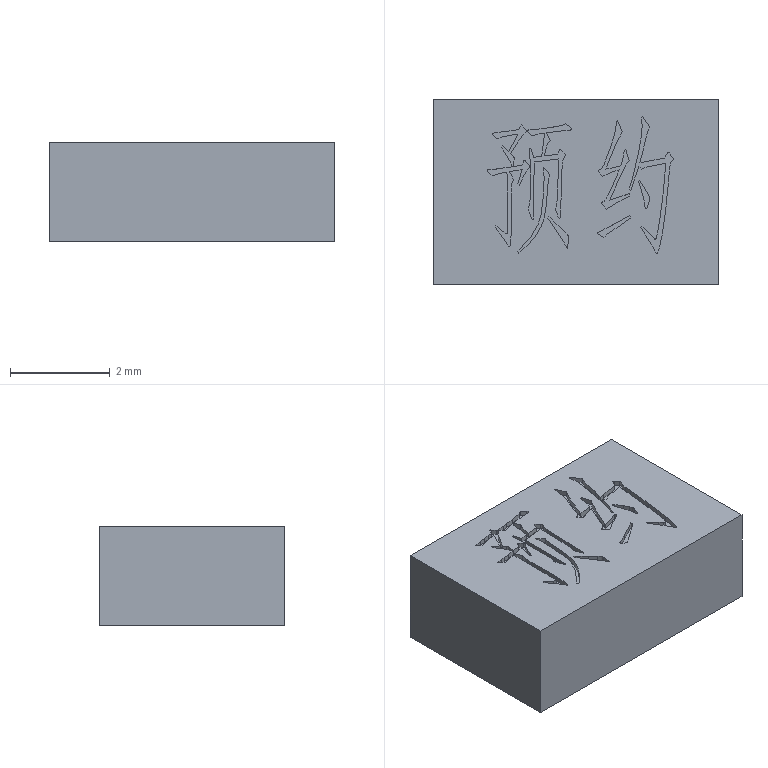Component | SolidWorks | Button4-1 | 1 solid | 206 faces | box 5.7 x 3.7 x 2 mm | volume 42 mm3 | plane 149 | spline 57
build123d program:
from build123d import *

# Parameters (mm, degrees)
SKETCH1_W           = 5.7
SKETCH1_H           = 3.7
BOSS_EXTRUDE1_DEPTH = 2
CUT_EXTRUDE1_DEPTH  = 0.1


with BuildPart() as part:
    # Sketch1 → Boss-Extrude1 (new body)
    with BuildSketch(Plane.XY):
        with Locations((2.85, 1.85)):
            Rectangle(SKETCH1_W, SKETCH1_H)
    extrude(amount=BOSS_EXTRUDE1_DEPTH)

    # Sketch2 → Cut-Extrude1 (cut)
    with BuildSketch(Plane.XY.offset(2)):
        with BuildLine():
            Line((1.574, 2.354), (1.551, 2.409))
            add(Edge.make_bspline(
                [(1.551, 2.409), (1.542, 2.43), (1.522, 2.474), (1.485, 2.54), (1.442, 2.612), (1.41, 2.66), (1.393, 2.685)],
                knots=[0, 0, 0, 0, 0.8687, 1.824, 2.865, 4, 4, 4, 4], degree=3))
            Line((1.393, 2.685), (1.359, 2.734))
            Line((1.359, 2.734), (1.373, 2.771))
            Line((1.373, 2.771), (1.396, 2.751))
            Line((1.396, 2.751), (1.505, 2.656))
            add(Edge.make_bspline(
                [(1.505, 2.656), (1.512, 2.667), (1.525, 2.69), (1.545, 2.727), (1.566, 2.766), (1.588, 2.808), (1.61, 2.854), (1.634, 2.902), (1.658, 2.953), (1.675, 2.989), (1.683, 3.007)],
                knots=[0, 0, 0, 0, 0.7801, 1.622, 2.525, 3.489, 4.524, 5.617, 6.775, 8, 8, 8, 8], degree=3))
            Line((1.683, 3.007), (1.577, 2.99))
            add(Edge.make_bspline(
                [(1.577, 2.99), (1.558, 2.987), (1.522, 2.98), (1.469, 2.97), (1.422, 2.961), (1.379, 2.952), (1.342, 2.942), (1.309, 2.933), (1.282, 2.924), (1.265, 2.918), (1.258, 2.915)],
                knots=[0, 0, 0, 0, 1.411, 2.709, 3.882, 4.944, 5.884, 6.704, 7.413, 8, 8, 8, 8], degree=3))
            Line((1.258, 2.915), (1.192, 2.987))
            add(Edge.make_bspline(
                [(1.192, 2.987), (1.186, 2.991), (1.178, 2.998), (1.172, 3.013), (1.179, 3.021), (1.189, 3.025), (1.204, 3.03), (1.216, 3.032), (1.223, 3.033)],
                knots=[0, 0, 0, 0, 1.454, 2.302, 2.76, 3.483, 4.56, 6, 6, 6, 6], degree=3))
            Line((1.223, 3.033), (1.353, 3.05))
            Line((1.353, 3.05), (1.485, 3.065))
            Line((1.485, 3.065), (1.591, 3.082))
            Line((1.591, 3.082), (1.701, 3.096))
            Line((1.701, 3.096), (1.741, 3.168))
            add(Edge.make_bspline(
                [(1.741, 3.168), (1.743, 3.172), (1.747, 3.179), (1.752, 3.187), (1.756, 3.192), (1.758, 3.196), (1.762, 3.194), (1.767, 3.19), (1.773, 3.183), (1.778, 3.177), (1.781, 3.174)],
                knots=[0, 0, 0, 0, 1.64, 2.878, 3.674, 4.05, 4.385, 5.107, 6.347, 8, 8, 8, 8], degree=3))
            Line((1.781, 3.174), (1.844, 3.099))
            add(Edge.make_bspline(
                [(1.844, 3.099), (1.849, 3.093), (1.855, 3.083), (1.859, 3.068), (1.855, 3.058), (1.849, 3.05), (1.839, 3.041), (1.821, 3.027), (1.795, 3.003), (1.773, 2.975), (1.754, 2.949), (1.739, 2.926), (1.718, 2.895), (1.693, 2.855), (1.662, 2.808), (1.625, 2.752), (1.585, 2.688), (1.555, 2.643), (1.54, 2.619)],
                knots=[0, 0, 0, 0, 0.5778, 0.9885, 1.187, 1.454, 1.816, 2.262, 3.348, 4.677, 5.177, 5.931, 6.952, 8.228, 9.781, 11.595, 13.664, 16, 16, 16, 16], degree=3))
            Line((1.54, 2.619), (1.597, 2.558))
            add(Edge.make_bspline(
                [(1.597, 2.558), (1.6, 2.554), (1.605, 2.546), (1.611, 2.537), (1.613, 2.529), (1.612, 2.519), (1.611, 2.506), (1.61, 2.495), (1.609, 2.489)],
                knots=[0, 0, 0, 0, 1.384, 2.211, 2.635, 3.368, 4.524, 6, 6, 6, 6], degree=3))
            Line((1.609, 2.489), (1.586, 2.357))
            Line((1.586, 2.357), (1.767, 2.383))
            Line((1.767, 2.383), (1.801, 2.461))
            add(Edge.make_bspline(
                [(1.801, 2.461), (1.804, 2.465), (1.807, 2.473), (1.82, 2.48), (1.834, 2.473), (1.84, 2.465), (1.844, 2.461)],
                knots=[0, 0, 0, 0, 1.058, 1.818, 2.714, 4, 4, 4, 4], degree=3))
            Line((1.844, 2.461), (1.896, 2.394))
            add(Edge.make_bspline(
                [(1.896, 2.394), (1.9, 2.389), (1.906, 2.379), (1.913, 2.367), (1.917, 2.357), (1.919, 2.349), (1.915, 2.342), (1.908, 2.332), (1.898, 2.32), (1.883, 2.305), (1.866, 2.284), (1.847, 2.256), (1.826, 2.22), (1.812, 2.193), (1.804, 2.179)],
                knots=[0, 0, 0, 0, 0.87, 1.559, 2.026, 2.348, 2.671, 3.202, 3.926, 4.901, 6.149, 7.717, 9.686, 12, 12, 12, 12], degree=3))
            Line((1.804, 2.179), (1.761, 2.081))
            Line((1.761, 2.081), (1.712, 1.977))
            Line((1.712, 1.977), (1.686, 2.009))
            Line((1.686, 2.009), (1.773, 2.297))
            Line((1.773, 2.297), (1.514, 2.256))
            Line((1.514, 2.256), (1.6, 2.106))
            add(Edge.make_bspline(
                [(1.6, 2.106), (1.596, 2.095), (1.587, 2.075), (1.576, 2.049), (1.57, 2.029), (1.565, 2.015), (1.564, 2), (1.563, 1.981), (1.561, 1.956), (1.56, 1.936), (1.56, 1.925)],
                knots=[0, 0, 0, 0, 1.554, 2.768, 3.652, 4.198, 4.709, 5.51, 6.619, 8, 8, 8, 8], degree=3))
            Line((1.56, 1.925), (1.554, 1.828))
            Line((1.554, 1.828), (1.551, 1.117))
            Line((1.551, 1.117), (1.551, 1.013))
            add(Edge.make_bspline(
                [(1.551, 1.013), (1.55, 0.9875), (1.548, 0.9319), (1.543, 0.8624), (1.538, 0.8088), (1.533, 0.778), (1.528, 0.7589), (1.519, 0.747), (1.509, 0.7499), (1.5, 0.7564), (1.49, 0.7675), (1.477, 0.7866), (1.464, 0.8099), (1.455, 0.8278), (1.451, 0.8352)],
                knots=[0, 0, 0, 0, 2.434, 5.233, 6.549, 7.511, 8.132, 8.453, 8.71, 9.047, 9.501, 10.086, 11.211, 12, 12, 12, 12], degree=3))
            Line((1.451, 0.8352), (1.353, 0.9818))
            Line((1.353, 0.9818), (1.232, 1.14))
            Line((1.232, 1.14), (1.246, 1.177))
            Line((1.246, 1.177), (1.405, 1.048))
            add(Edge.make_bspline(
                [(1.405, 1.048), (1.412, 1.042), (1.423, 1.032), (1.44, 1.021), (1.452, 1.014), (1.463, 1.014), (1.469, 1.023), (1.471, 1.036), (1.473, 1.055), (1.472, 1.089), (1.471, 1.139), (1.473, 1.207), (1.476, 1.281), (1.478, 1.332), (1.479, 1.359)],
                knots=[0, 0, 0, 0, 0.7812, 1.36, 1.741, 1.977, 2.215, 2.595, 3.128, 3.832, 5.549, 7.538, 9.714, 12, 12, 12, 12], degree=3))
            Line((1.479, 1.359), (1.482, 1.848))
            add(Edge.make_bspline(
                [(1.482, 1.848), (1.482, 1.869), (1.482, 1.907), (1.482, 1.962), (1.482, 2.008), (1.481, 2.047), (1.48, 2.079), (1.479, 2.105), (1.479, 2.126), (1.478, 2.143), (1.476, 2.16), (1.473, 2.183), (1.47, 2.211), (1.467, 2.233), (1.465, 2.245)],
                knots=[0, 0, 0, 0, 1.878, 3.511, 4.913, 6.071, 7.023, 7.82, 8.438, 8.889, 9.366, 10.039, 10.921, 12, 12, 12, 12], degree=3))
            Line((1.465, 2.245), (1.353, 2.228))
            add(Edge.make_bspline(
                [(1.353, 2.228), (1.321, 2.221), (1.258, 2.208), (1.199, 2.185), (1.169, 2.173)],
                knots=[0, 0, 0, 0, 0.9976, 2, 2, 2, 2], degree=3))
            Line((1.169, 2.173), (1.083, 2.256))
            add(Edge.make_bspline(
                [(1.083, 2.256), (1.078, 2.26), (1.071, 2.267), (1.069, 2.283), (1.085, 2.292), (1.096, 2.293), (1.103, 2.294)],
                knots=[0, 0, 0, 0, 1.139, 1.841, 2.65, 4, 4, 4, 4], degree=3))
            Line((1.103, 2.294), (1.192, 2.302))
            Line((1.192, 2.302), (1.284, 2.311))
            Line((1.284, 2.311), (1.428, 2.334))
            Line((1.428, 2.334), (1.574, 2.354))
        make_face()
        with BuildLine():
            Line((1.681, 0.6656), (1.715, 0.7001))
            add(Edge.make_bspline(
                [(1.715, 0.7001), (1.734, 0.7193), (1.769, 0.7556), (1.819, 0.8079), (1.862, 0.855), (1.901, 0.898), (1.938, 0.9442), (1.975, 0.9977), (2.014, 1.061), (2.054, 1.131), (2.092, 1.205), (2.123, 1.282), (2.145, 1.357), (2.159, 1.434), (2.168, 1.514), (2.178, 1.598), (2.188, 1.689), (2.197, 1.784), (2.205, 1.88), (2.21, 1.971), (2.213, 2.055), (2.213, 2.109), (2.213, 2.135)],
                knots=[0, 0, 0, 0, 1.017, 1.931, 2.738, 3.443, 4.154, 4.978, 5.915, 6.968, 8.056, 9.097, 10.095, 11.063, 12.06, 13.137, 14.301, 15.539, 16.781, 17.94, 19.011, 20, 20, 20, 20], degree=3))
            add(Edge.make_bspline(
                [(2.213, 2.135), (2.212, 2.147), (2.212, 2.169), (2.209, 2.199), (2.208, 2.225), (2.205, 2.241), (2.204, 2.248)],
                knots=[0, 0, 0, 0, 1.244, 2.322, 3.25, 4, 4, 4, 4], degree=3))
            Line((2.204, 2.248), (2.196, 2.311))
            Line((2.196, 2.311), (2.204, 2.343))
            Line((2.204, 2.343), (2.325, 2.196))
            add(Edge.make_bspline(
                [(2.325, 2.196), (2.322, 2.187), (2.315, 2.17), (2.306, 2.143), (2.299, 2.111), (2.294, 2.083), (2.292, 2.058), (2.29, 2.04), (2.288, 2.018), (2.287, 1.992), (2.285, 1.962), (2.283, 1.928), (2.281, 1.89), (2.278, 1.833), (2.274, 1.757), (2.265, 1.663), (2.254, 1.564), (2.241, 1.463), (2.223, 1.362), (2.195, 1.264), (2.16, 1.171), (2.115, 1.084), (2.066, 1.003), (2.014, 0.9282), (1.96, 0.8607), (1.904, 0.802), (1.851, 0.7519), (1.806, 0.7092), (1.768, 0.6751), (1.745, 0.6563), (1.735, 0.6481)],
                knots=[0, 0, 0, 0, 0.4735, 0.8985, 1.382, 2.069, 2.292, 2.584, 2.945, 3.369, 3.855, 4.41, 5.034, 5.721, 7.193, 8.737, 10.347, 12.024, 13.709, 15.35, 16.968, 18.567, 20.121, 21.589, 22.993, 24.326, 25.536, 26.551, 27.37, 28, 28, 28, 28], degree=3))
            Line((1.735, 0.6481), (1.701, 0.6221))
            Line((1.701, 0.6221), (1.681, 0.6656))
        make_face()
        with BuildLine():
            Line((2.15, 3.114), (2.334, 3.14))
            add(Edge.make_bspline(
                [(2.334, 3.14), (2.353, 3.142), (2.388, 3.148), (2.438, 3.156), (2.482, 3.163), (2.519, 3.17), (2.55, 3.178), (2.575, 3.184), (2.593, 3.19), (2.603, 3.195), (2.607, 3.197)],
                knots=[0, 0, 0, 0, 1.638, 3.081, 4.354, 5.434, 6.346, 7.076, 7.619, 8, 8, 8, 8], degree=3))
            Line((2.607, 3.197), (2.647, 3.22))
            Line((2.647, 3.22), (2.748, 3.137))
            add(Edge.make_bspline(
                [(2.748, 3.137), (2.753, 3.131), (2.763, 3.123), (2.769, 3.108), (2.766, 3.097), (2.758, 3.093), (2.747, 3.089), (2.739, 3.088), (2.733, 3.088)],
                knots=[0, 0, 0, 0, 1.676, 2.889, 3.395, 3.99, 4.869, 6, 6, 6, 6], degree=3))
            Line((2.733, 3.088), (2.48, 3.062))
            Line((2.48, 3.062), (2.256, 3.033))
            Line((2.256, 3.033), (2.331, 2.889))
            add(Edge.make_bspline(
                [(2.331, 2.889), (2.323, 2.879), (2.306, 2.856), (2.287, 2.828), (2.273, 2.804), (2.267, 2.785), (2.259, 2.761), (2.251, 2.733), (2.243, 2.699), (2.235, 2.66), (2.227, 2.617), (2.221, 2.586), (2.219, 2.57)],
                knots=[0, 0, 0, 0, 1.092, 2.497, 2.946, 3.532, 4.25, 5.111, 6.12, 7.273, 8.563, 10, 10, 10, 10], degree=3))
            Line((2.219, 2.57), (2.486, 2.604))
            Line((2.486, 2.604), (2.512, 2.679))
            add(Edge.make_bspline(
                [(2.512, 2.679), (2.514, 2.684), (2.518, 2.693), (2.525, 2.703), (2.534, 2.708), (2.539, 2.704), (2.541, 2.702)],
                knots=[0, 0, 0, 0, 1.53, 2.568, 3.261, 4, 4, 4, 4], degree=3))
            Line((2.541, 2.702), (2.613, 2.624))
            add(Edge.make_bspline(
                [(2.613, 2.624), (2.619, 2.617), (2.629, 2.605), (2.639, 2.585), (2.634, 2.565), (2.626, 2.553), (2.621, 2.547)],
                knots=[0, 0, 0, 0, 1.29, 2.137, 2.904, 4, 4, 4, 4], degree=3))
            add(Edge.make_bspline(
                [(2.621, 2.547), (2.614, 2.536), (2.601, 2.516), (2.588, 2.489), (2.581, 2.464), (2.577, 2.442), (2.574, 2.415), (2.573, 2.396), (2.572, 2.386)],
                knots=[0, 0, 0, 0, 1.308, 2.536, 3.188, 3.978, 4.923, 6, 6, 6, 6], degree=3))
            Line((2.572, 2.386), (2.549, 1.687))
            add(Edge.make_bspline(
                [(2.549, 1.687), (2.549, 1.663), (2.547, 1.62), (2.545, 1.561), (2.544, 1.515), (2.542, 1.48), (2.541, 1.449), (2.539, 1.417), (2.535, 1.382), (2.533, 1.352), (2.53, 1.329), (2.527, 1.318), (2.523, 1.309), (2.515, 1.31), (2.51, 1.317), (2.504, 1.329), (2.496, 1.346), (2.491, 1.36), (2.489, 1.368)],
                knots=[0, 0, 0, 0, 2.539, 4.638, 6.264, 7.451, 8.454, 9.581, 10.848, 12.222, 12.837, 13.265, 13.526, 13.693, 13.994, 14.464, 15.13, 16, 16, 16, 16], degree=3))
            Line((2.489, 1.368), (2.454, 1.465))
            add(Edge.make_bspline(
                [(2.454, 1.465), (2.452, 1.472), (2.448, 1.484), (2.443, 1.499), (2.439, 1.51), (2.438, 1.519), (2.445, 1.532), (2.451, 1.554), (2.46, 1.586), (2.466, 1.623), (2.471, 1.659), (2.476, 1.687), (2.478, 1.71), (2.48, 1.731), (2.48, 1.757), (2.48, 1.777), (2.48, 1.787)],
                knots=[0, 0, 0, 0, 0.9227, 1.61, 2.081, 2.299, 2.815, 3.846, 5.275, 6.985, 8.668, 9.952, 10.626, 11.517, 12.641, 14, 14, 14, 14], degree=3))
            Line((2.48, 1.787), (2.489, 2.069))
            Line((2.489, 2.069), (2.5, 2.509))
            Line((2.5, 2.509), (2.012, 2.449))
            Line((2.012, 2.449), (2.003, 1.557))
            Line((2.003, 1.557), (2, 1.353))
            add(Edge.make_bspline(
                [(2, 1.353), (2, 1.346), (2, 1.335), (1.998, 1.319), (1.996, 1.308), (1.991, 1.299), (1.984, 1.293), (1.975, 1.293), (1.971, 1.299), (1.967, 1.307), (1.962, 1.319), (1.959, 1.328), (1.957, 1.333)],
                knots=[0, 0, 0, 0, 1.685, 3.012, 3.999, 4.703, 5.59, 6.251, 6.743, 7.53, 8.598, 10, 10, 10, 10], degree=3))
            Line((1.957, 1.333), (1.914, 1.442))
            add(Edge.make_bspline(
                [(1.914, 1.442), (1.91, 1.45), (1.903, 1.464), (1.896, 1.482), (1.891, 1.494), (1.889, 1.502), (1.891, 1.507), (1.893, 1.515), (1.897, 1.525), (1.905, 1.543), (1.914, 1.573), (1.921, 1.616), (1.928, 1.661), (1.931, 1.708), (1.934, 1.76), (1.936, 1.796), (1.937, 1.816)],
                knots=[0, 0, 0, 0, 0.9721, 1.681, 2.148, 2.367, 2.529, 2.809, 3.207, 3.708, 5.009, 6.634, 8.387, 10.007, 11.795, 14, 14, 14, 14], degree=3))
            Line((1.937, 1.816), (1.937, 2.394))
            add(Edge.make_bspline(
                [(1.937, 2.394), (1.937, 2.395), (1.937, 2.398), (1.937, 2.405), (1.937, 2.416), (1.937, 2.432), (1.936, 2.452), (1.936, 2.478), (1.934, 2.508), (1.932, 2.558), (1.927, 2.628), (1.92, 2.686), (1.917, 2.716)],
                knots=[0, 0, 0, 0, 0.06597, 0.2771, 0.6201, 1.108, 1.742, 2.547, 3.485, 4.594, 7.134, 10, 10, 10, 10], degree=3))
            Line((1.917, 2.716), (1.945, 2.728))
            Line((1.945, 2.728), (2.003, 2.541))
            Line((2.003, 2.541), (2.164, 2.564))
            add(Edge.make_bspline(
                [(2.164, 2.564), (2.167, 2.581), (2.172, 2.612), (2.179, 2.651), (2.184, 2.686), (2.189, 2.719), (2.193, 2.762), (2.199, 2.81), (2.204, 2.856), (2.207, 2.895), (2.209, 2.923), (2.21, 2.938), (2.21, 2.944)],
                knots=[0, 0, 0, 0, 1.298, 2.473, 3.138, 4.037, 5.146, 6.49, 7.8, 8.828, 9.554, 10, 10, 10, 10], degree=3))
            Line((2.21, 2.944), (2.213, 3.027))
            add(Edge.make_bspline(
                [(2.213, 3.027), (2.189, 3.024), (2.144, 3.018), (2.08, 3.005), (2.022, 2.99), (1.986, 2.976), (1.969, 2.969)],
                knots=[0, 0, 0, 0, 1.129, 2.166, 3.121, 4, 4, 4, 4], degree=3))
            Line((1.969, 2.969), (1.891, 3.047))
            add(Edge.make_bspline(
                [(1.891, 3.047), (1.887, 3.052), (1.88, 3.059), (1.874, 3.071), (1.876, 3.08), (1.883, 3.084), (1.894, 3.088), (1.903, 3.089), (1.908, 3.091)],
                knots=[0, 0, 0, 0, 1.498, 2.59, 3.084, 3.731, 4.696, 6, 6, 6, 6], degree=3))
            Line((1.908, 3.091), (2.038, 3.102))
            Line((2.038, 3.102), (2.15, 3.114))
        make_face()
        with BuildLine():
            Line((2.285, 1.327), (2.305, 1.365))
            Line((2.305, 1.365), (2.36, 1.31))
            Line((2.36, 1.31), (2.512, 1.16))
            Line((2.512, 1.16), (2.647, 1.028))
            add(Edge.make_bspline(
                [(2.647, 1.028), (2.653, 1.022), (2.663, 1.011), (2.676, 0.9954), (2.686, 0.9836), (2.695, 0.9711), (2.701, 0.9521), (2.7, 0.9364), (2.699, 0.9273)],
                knots=[0, 0, 0, 0, 1.256, 2.285, 3.069, 3.615, 4.615, 6, 6, 6, 6], degree=3))
            Line((2.699, 0.9273), (2.687, 0.7777))
            add(Edge.make_bspline(
                [(2.687, 0.7777), (2.687, 0.7717), (2.686, 0.7612), (2.685, 0.7477), (2.684, 0.7388), (2.684, 0.7328), (2.68, 0.7288), (2.675, 0.7256), (2.668, 0.7315), (2.661, 0.7416), (2.652, 0.759), (2.645, 0.7727), (2.641, 0.7807)],
                knots=[0, 0, 0, 0, 1.5, 2.645, 3.397, 3.76, 4.117, 4.659, 5.124, 6.143, 7.769, 10, 10, 10, 10], degree=3))
            Line((2.641, 0.7807), (2.601, 0.8523))
            add(Edge.make_bspline(
                [(2.601, 0.8523), (2.594, 0.8651), (2.579, 0.8922), (2.553, 0.9347), (2.523, 0.9812), (2.49, 1.033), (2.453, 1.088), (2.412, 1.148), (2.367, 1.211), (2.335, 1.255), (2.319, 1.278)],
                knots=[0, 0, 0, 0, 0.6936, 1.466, 2.336, 3.291, 4.335, 5.467, 6.689, 8, 8, 8, 8], degree=3))
            Line((2.319, 1.278), (2.285, 1.327))
        make_face()
        with BuildLine():
            Line((3.915, 1.905), (3.929, 1.954))
            Line((3.929, 1.954), (3.969, 2.083))
            add(Edge.make_bspline(
                [(3.969, 2.083), (3.972, 2.092), (3.977, 2.11), (3.985, 2.14), (3.993, 2.174), (4.003, 2.212), (4.013, 2.255), (4.025, 2.302), (4.037, 2.354), (4.05, 2.409), (4.063, 2.463), (4.075, 2.515), (4.085, 2.563), (4.095, 2.606), (4.103, 2.645), (4.111, 2.68), (4.117, 2.71), (4.126, 2.761), (4.138, 2.835), (4.151, 2.915), (4.16, 2.976), (4.165, 3.016), (4.17, 3.049), (4.173, 3.086), (4.176, 3.127), (4.176, 3.158), (4.176, 3.174)],
                knots=[0, 0, 0, 0, 0.5622, 1.229, 1.988, 2.842, 3.788, 4.838, 5.983, 7.23, 8.477, 9.619, 10.675, 11.634, 12.491, 13.261, 13.927, 14.506, 16.624, 18.747, 19.751, 20.614, 21.346, 21.946, 22.988, 24, 24, 24, 24], degree=3))
            add(Edge.make_bspline(
                [(4.176, 3.174), (4.176, 3.186), (4.174, 3.21), (4.17, 3.248), (4.164, 3.289), (4.159, 3.317), (4.156, 3.332)],
                knots=[0, 0, 0, 0, 0.8682, 1.824, 2.872, 4, 4, 4, 4], degree=3))
            Line((4.156, 3.332), (4.176, 3.361))
            Line((4.176, 3.361), (4.326, 3.154))
            add(Edge.make_bspline(
                [(4.326, 3.154), (4.319, 3.139), (4.306, 3.112), (4.29, 3.071), (4.276, 3.033), (4.265, 2.995), (4.256, 2.957), (4.246, 2.914), (4.234, 2.867), (4.223, 2.816), (4.211, 2.765), (4.2, 2.719), (4.191, 2.678), (4.185, 2.653), (4.182, 2.642)],
                knots=[0, 0, 0, 0, 1.078, 2.063, 2.979, 3.817, 4.676, 5.654, 6.759, 7.981, 9.193, 10.266, 11.202, 12, 12, 12, 12], degree=3))
            Line((4.182, 2.642), (4.145, 2.498))
            Line((4.145, 2.498), (4.13, 2.438))
            Line((4.13, 2.438), (4.243, 2.455))
            Line((4.243, 2.455), (4.619, 2.527))
            Line((4.619, 2.527), (4.674, 2.624))
            add(Edge.make_bspline(
                [(4.674, 2.624), (4.678, 2.63), (4.683, 2.64), (4.697, 2.648), (4.713, 2.643), (4.719, 2.635), (4.723, 2.63)],
                knots=[0, 0, 0, 0, 1.227, 2.09, 2.863, 4, 4, 4, 4], degree=3))
            Line((4.723, 2.63), (4.78, 2.544))
            add(Edge.make_bspline(
                [(4.78, 2.544), (4.783, 2.54), (4.788, 2.532), (4.793, 2.522), (4.796, 2.514), (4.797, 2.508), (4.793, 2.502), (4.789, 2.495), (4.781, 2.485), (4.768, 2.469), (4.753, 2.45), (4.742, 2.429), (4.737, 2.41), (4.733, 2.391), (4.73, 2.364), (4.727, 2.345), (4.726, 2.334)],
                knots=[0, 0, 0, 0, 0.9006, 1.591, 2.08, 2.39, 2.701, 3.244, 3.98, 4.949, 6.88, 8.376, 9.207, 10.414, 12.027, 14, 14, 14, 14], degree=3))
            Line((4.726, 2.334), (4.711, 2.176))
            Line((4.711, 2.176), (4.688, 1.922))
            Line((4.688, 1.922), (4.657, 1.609))
            Line((4.657, 1.609), (4.625, 1.336))
            Line((4.625, 1.336), (4.608, 1.215))
            Line((4.608, 1.215), (4.585, 1.051))
            add(Edge.make_bspline(
                [(4.585, 1.051), (4.583, 1.038), (4.577, 1.009), (4.568, 0.9614), (4.557, 0.9029), (4.545, 0.849), (4.536, 0.8039), (4.529, 0.7724), (4.523, 0.7441), (4.516, 0.7193), (4.511, 0.6976), (4.505, 0.6797), (4.501, 0.6647), (4.495, 0.6504), (4.489, 0.6366), (4.481, 0.624), (4.475, 0.6156), (4.469, 0.6109), (4.462, 0.6136), (4.456, 0.6207), (4.45, 0.6313), (4.446, 0.6401), (4.444, 0.6452)],
                knots=[0, 0, 0, 0, 1.538, 3.495, 5.869, 8.664, 10.088, 11.375, 12.526, 13.561, 14.439, 15.203, 15.811, 16.307, 17.06, 17.631, 18.043, 18.294, 18.525, 18.85, 19.346, 20, 20, 20, 20], degree=3))
            Line((4.444, 0.6452), (4.392, 0.7432))
            Line((4.392, 0.7432), (4.323, 0.8612))
            Line((4.323, 0.8612), (4.15, 1.134))
            Line((4.15, 1.134), (4.171, 1.166))
            Line((4.171, 1.166), (4.263, 1.074))
            Line((4.263, 1.074), (4.343, 0.9933))
            Line((4.343, 0.9933), (4.401, 0.9328))
            add(Edge.make_bspline(
                [(4.401, 0.9328), (4.405, 0.9286), (4.411, 0.921), (4.422, 0.9128), (4.429, 0.9068), (4.438, 0.9046), (4.446, 0.9096), (4.454, 0.9203), (4.459, 0.9384), (4.462, 0.953), (4.464, 0.9618)],
                knots=[0, 0, 0, 0, 1.23, 2.183, 2.844, 3.281, 3.99, 4.796, 6.06, 8, 8, 8, 8], degree=3))
            Line((4.464, 0.9618), (4.481, 1.028))
            Line((4.481, 1.028), (4.504, 1.149))
            Line((4.504, 1.149), (4.53, 1.31))
            Line((4.53, 1.31), (4.562, 1.557))
            Line((4.562, 1.557), (4.591, 1.787))
            Line((4.591, 1.787), (4.614, 2.043))
            Line((4.614, 2.043), (4.637, 2.291))
            Line((4.637, 2.291), (4.645, 2.423))
            add(Edge.make_bspline(
                [(4.645, 2.423), (4.622, 2.418), (4.575, 2.408), (4.508, 2.395), (4.445, 2.384), (4.384, 2.374), (4.326, 2.364), (4.27, 2.349), (4.215, 2.332), (4.18, 2.316), (4.162, 2.308)],
                knots=[0, 0, 0, 0, 1.168, 2.269, 3.304, 4.275, 5.208, 6.134, 7.065, 8, 8, 8, 8], degree=3))
            Line((4.162, 2.308), (4.107, 2.36))
            add(Edge.make_bspline(
                [(4.107, 2.36), (4.101, 2.339), (4.088, 2.299), (4.07, 2.242), (4.053, 2.19), (4.038, 2.145), (4.025, 2.104), (4.013, 2.07), (4.004, 2.041), (3.993, 2.011), (3.983, 1.982), (3.973, 1.954), (3.966, 1.934), (3.962, 1.924), (3.961, 1.92)],
                knots=[0, 0, 0, 0, 1.702, 3.255, 4.646, 5.899, 6.99, 7.932, 8.724, 9.366, 10.371, 11.141, 11.693, 12, 12, 12, 12], degree=3))
            Line((3.961, 1.92), (3.949, 1.879))
            Line((3.949, 1.879), (3.915, 1.905))
        make_face()
        with BuildLine():
            Line((4.101, 2.055), (4.122, 2.086))
            Line((4.122, 2.086), (4.15, 2.046))
            Line((4.15, 2.046), (4.24, 1.905))
            Line((4.24, 1.905), (4.309, 1.782))
            add(Edge.make_bspline(
                [(4.309, 1.782), (4.313, 1.771), (4.32, 1.753), (4.328, 1.727), (4.329, 1.7), (4.323, 1.684), (4.32, 1.675)],
                knots=[0, 0, 0, 0, 1.204, 2.145, 2.991, 4, 4, 4, 4], degree=3))
            Line((4.32, 1.675), (4.272, 1.534))
            add(Edge.make_bspline(
                [(4.272, 1.534), (4.269, 1.528), (4.266, 1.519), (4.257, 1.507), (4.244, 1.509), (4.24, 1.516), (4.237, 1.52)],
                knots=[0, 0, 0, 0, 1.411, 2.275, 2.954, 4, 4, 4, 4], degree=3))
            Line((4.237, 1.52), (4.225, 1.606))
            Line((4.225, 1.606), (4.197, 1.753))
            add(Edge.make_bspline(
                [(4.197, 1.753), (4.195, 1.761), (4.19, 1.78), (4.183, 1.808), (4.174, 1.841), (4.163, 1.877), (4.15, 1.916), (4.135, 1.96), (4.119, 2.006), (4.107, 2.038), (4.101, 2.055)],
                knots=[0, 0, 0, 0, 0.6627, 1.419, 2.268, 3.224, 4.265, 5.411, 6.663, 8, 8, 8, 8], degree=3))
        make_face()
        with BuildLine():
            add(Edge.make_bspline(
                [(3.446, 2.305), (3.469, 2.31), (3.516, 2.319), (3.59, 2.334), (3.666, 2.352), (3.718, 2.365), (3.745, 2.371)],
                knots=[0, 0, 0, 0, 0.9252, 1.903, 2.925, 4, 4, 4, 4], degree=3))
            Line((3.745, 2.371), (3.774, 2.458))
            add(Edge.make_bspline(
                [(3.774, 2.458), (3.775, 2.462), (3.778, 2.472), (3.781, 2.49), (3.787, 2.512), (3.792, 2.538), (3.798, 2.563), (3.802, 2.584), (3.806, 2.599), (3.808, 2.607), (3.808, 2.61)],
                knots=[0, 0, 0, 0, 0.6556, 1.592, 2.776, 4.225, 5.653, 6.747, 7.53, 8, 8, 8, 8], degree=3))
            Line((3.808, 2.61), (3.814, 2.688))
            Line((3.814, 2.688), (3.846, 2.702))
            Line((3.846, 2.702), (3.915, 2.478))
            add(Edge.make_bspline(
                [(3.915, 2.478), (3.907, 2.469), (3.89, 2.45), (3.866, 2.414), (3.84, 2.37), (3.817, 2.326), (3.795, 2.282), (3.774, 2.237), (3.748, 2.181), (3.717, 2.114), (3.681, 2.036), (3.641, 1.947), (3.595, 1.848), (3.563, 1.778), (3.547, 1.741)],
                knots=[0, 0, 0, 0, 0.5007, 1.119, 1.87, 2.737, 3.289, 4.018, 4.913, 5.986, 7.233, 8.65, 10.239, 12, 12, 12, 12], degree=3))
            Line((3.547, 1.741), (3.521, 1.684))
            Line((3.521, 1.684), (3.915, 1.816))
            Line((3.915, 1.816), (3.926, 1.767))
            add(Edge.make_bspline(
                [(3.926, 1.767), (3.907, 1.758), (3.867, 1.738), (3.804, 1.706), (3.734, 1.668), (3.671, 1.636), (3.622, 1.609), (3.587, 1.589), (3.556, 1.572), (3.529, 1.555), (3.505, 1.54), (3.486, 1.527), (3.47, 1.514), (3.461, 1.506), (3.457, 1.503)],
                knots=[0, 0, 0, 0, 1.407, 2.992, 4.759, 6.701, 7.672, 8.55, 9.348, 10.05, 10.668, 11.199, 11.644, 12, 12, 12, 12], degree=3))
            Line((3.457, 1.503), (3.371, 1.6))
            add(Edge.make_bspline(
                [(3.371, 1.6), (3.367, 1.605), (3.36, 1.613), (3.359, 1.63), (3.371, 1.645), (3.392, 1.653), (3.418, 1.667), (3.437, 1.686), (3.45, 1.705), (3.46, 1.721), (3.472, 1.744), (3.487, 1.771), (3.503, 1.804), (3.521, 1.844), (3.542, 1.888), (3.571, 1.954), (3.608, 2.036), (3.648, 2.129), (3.684, 2.213), (3.706, 2.266), (3.716, 2.291)],
                knots=[0, 0, 0, 0, 0.3961, 0.7243, 1.091, 1.579, 2.244, 3.077, 3.374, 3.816, 4.386, 5.094, 5.931, 6.911, 8.029, 9.277, 11.8, 14.104, 16.161, 18, 18, 18, 18], degree=3))
            add(Edge.make_bspline(
                [(3.716, 2.291), (3.69, 2.284), (3.636, 2.27), (3.554, 2.24), (3.47, 2.206), (3.414, 2.178), (3.386, 2.164)],
                knots=[0, 0, 0, 0, 0.9218, 1.894, 2.919, 4, 4, 4, 4], degree=3))
            Line((3.386, 2.164), (3.305, 2.251))
            add(Edge.make_bspline(
                [(3.305, 2.251), (3.301, 2.254), (3.294, 2.261), (3.293, 2.274), (3.299, 2.282), (3.306, 2.288), (3.316, 2.293), (3.33, 2.296), (3.344, 2.302), (3.358, 2.311), (3.371, 2.324), (3.382, 2.341), (3.394, 2.364), (3.408, 2.395), (3.424, 2.435), (3.442, 2.484), (3.464, 2.541), (3.488, 2.607), (3.516, 2.681), (3.546, 2.761), (3.576, 2.841), (3.601, 2.915), (3.62, 2.981), (3.632, 3.04), (3.641, 3.089), (3.647, 3.129), (3.652, 3.159), (3.652, 3.176), (3.653, 3.183)],
                knots=[0, 0, 0, 0, 0.3905, 0.7033, 0.8918, 1.114, 1.403, 1.768, 2.164, 2.577, 3.019, 3.506, 4.133, 4.987, 6.08, 7.393, 8.945, 10.725, 12.73, 14.964, 17.191, 19.178, 20.925, 22.426, 23.697, 24.71, 25.482, 26, 26, 26, 26], degree=3))
            Line((3.653, 3.183), (3.653, 3.266))
            Line((3.653, 3.266), (3.679, 3.286))
            Line((3.679, 3.286), (3.777, 3.053))
            add(Edge.make_bspline(
                [(3.777, 3.053), (3.772, 3.046), (3.762, 3.032), (3.747, 3.009), (3.732, 2.982), (3.716, 2.952), (3.699, 2.92), (3.683, 2.883), (3.664, 2.844), (3.647, 2.803), (3.629, 2.762), (3.614, 2.725), (3.6, 2.691), (3.587, 2.661), (3.577, 2.635), (3.568, 2.614), (3.561, 2.596), (3.557, 2.586), (3.555, 2.581)],
                knots=[0, 0, 0, 0, 0.7498, 1.594, 2.541, 3.57, 4.697, 5.923, 7.244, 8.653, 10.045, 11.303, 12.421, 13.41, 14.259, 14.979, 15.554, 16, 16, 16, 16], degree=3))
            Line((3.555, 2.581), (3.472, 2.374))
            Line((3.472, 2.374), (3.446, 2.305))
        make_face()
        with BuildLine():
            Line((3.929, 1.376), (3.94, 1.327))
            add(Edge.make_bspline(
                [(3.94, 1.327), (3.913, 1.309), (3.86, 1.273), (3.783, 1.219), (3.708, 1.168), (3.65, 1.126), (3.606, 1.095), (3.578, 1.074), (3.553, 1.057), (3.532, 1.042), (3.515, 1.03), (3.502, 1.02), (3.493, 1.013), (3.488, 1.009), (3.486, 1.008)],
                knots=[0, 0, 0, 0, 2.123, 4.161, 6.113, 7.976, 8.835, 9.587, 10.241, 10.788, 11.243, 11.598, 11.849, 12, 12, 12, 12], degree=3))
            Line((3.486, 1.008), (3.434, 0.9673))
            Line((3.434, 0.9673), (3.4, 0.9418))
            Line((3.4, 0.9418), (3.296, 1.002))
            add(Edge.make_bspline(
                [(3.296, 1.002), (3.292, 1.005), (3.284, 1.011), (3.283, 1.026), (3.285, 1.039), (3.292, 1.048), (3.3, 1.052), (3.309, 1.055), (3.322, 1.06), (3.335, 1.065), (3.348, 1.07), (3.362, 1.076), (3.38, 1.084), (3.4, 1.094), (3.425, 1.106), (3.452, 1.121), (3.484, 1.137), (3.506, 1.148), (3.518, 1.154)],
                knots=[0, 0, 0, 0, 0.7823, 1.539, 2.257, 2.817, 3.181, 3.718, 4.418, 5.303, 5.882, 6.691, 7.711, 8.943, 10.376, 12.032, 13.91, 16, 16, 16, 16], degree=3))
            Line((3.518, 1.154), (3.929, 1.376))
        make_face()
    extrude(amount=-CUT_EXTRUDE1_DEPTH, mode=Mode.SUBTRACT)


solid = part.part

# Placed as in the assembly
solid = solid.moved(Location((-69.806, -4.714, 277.152), (0, 0, 0)))